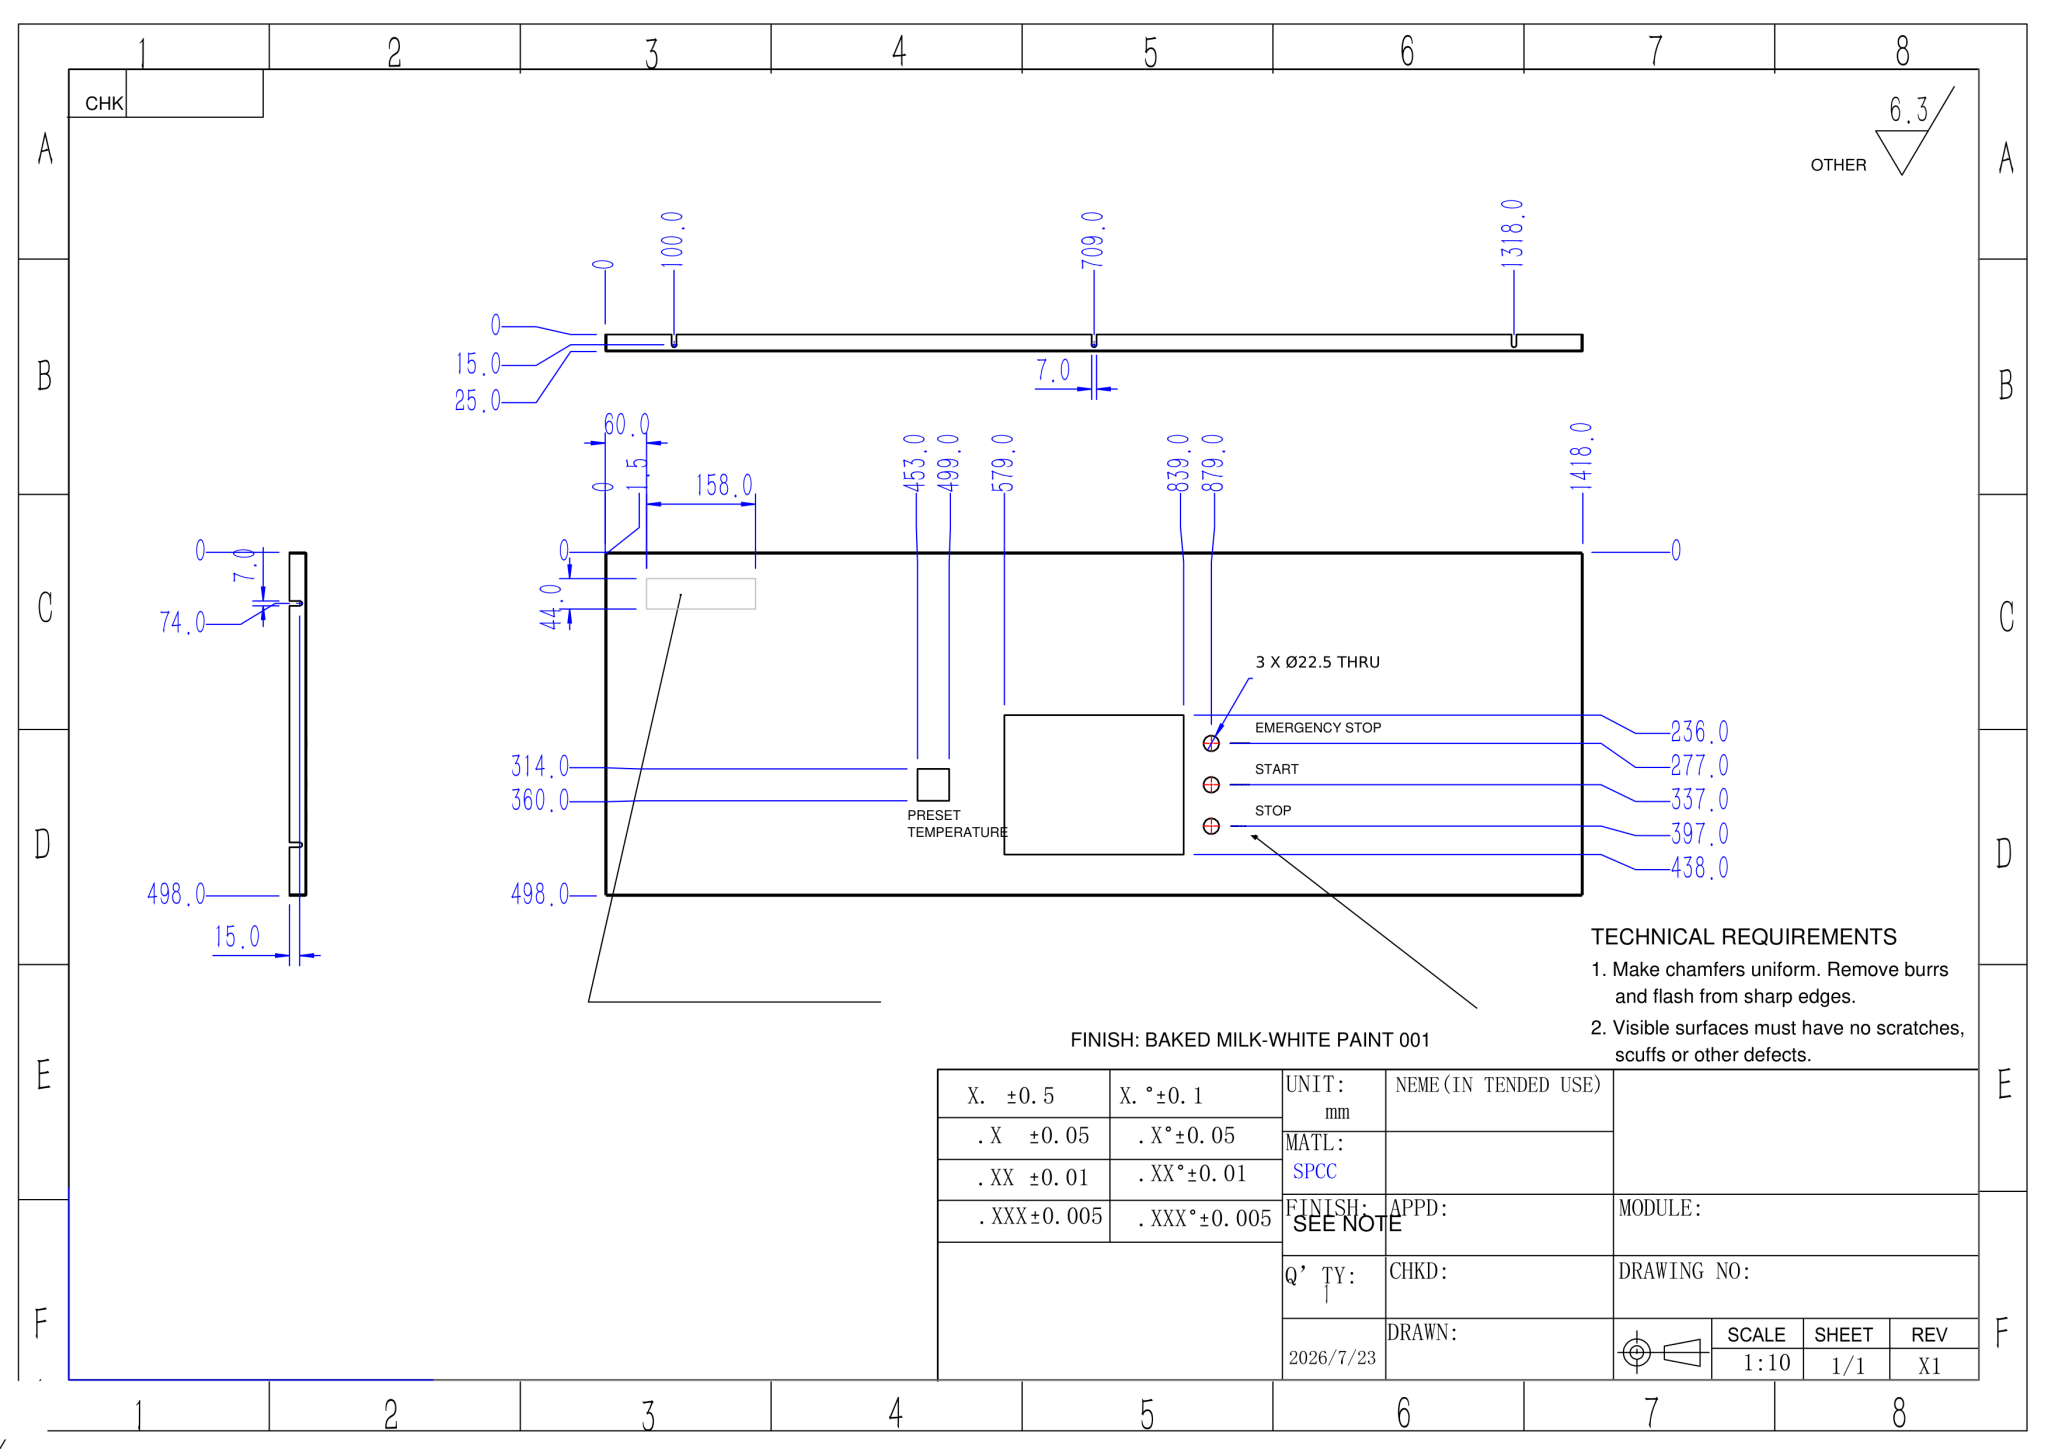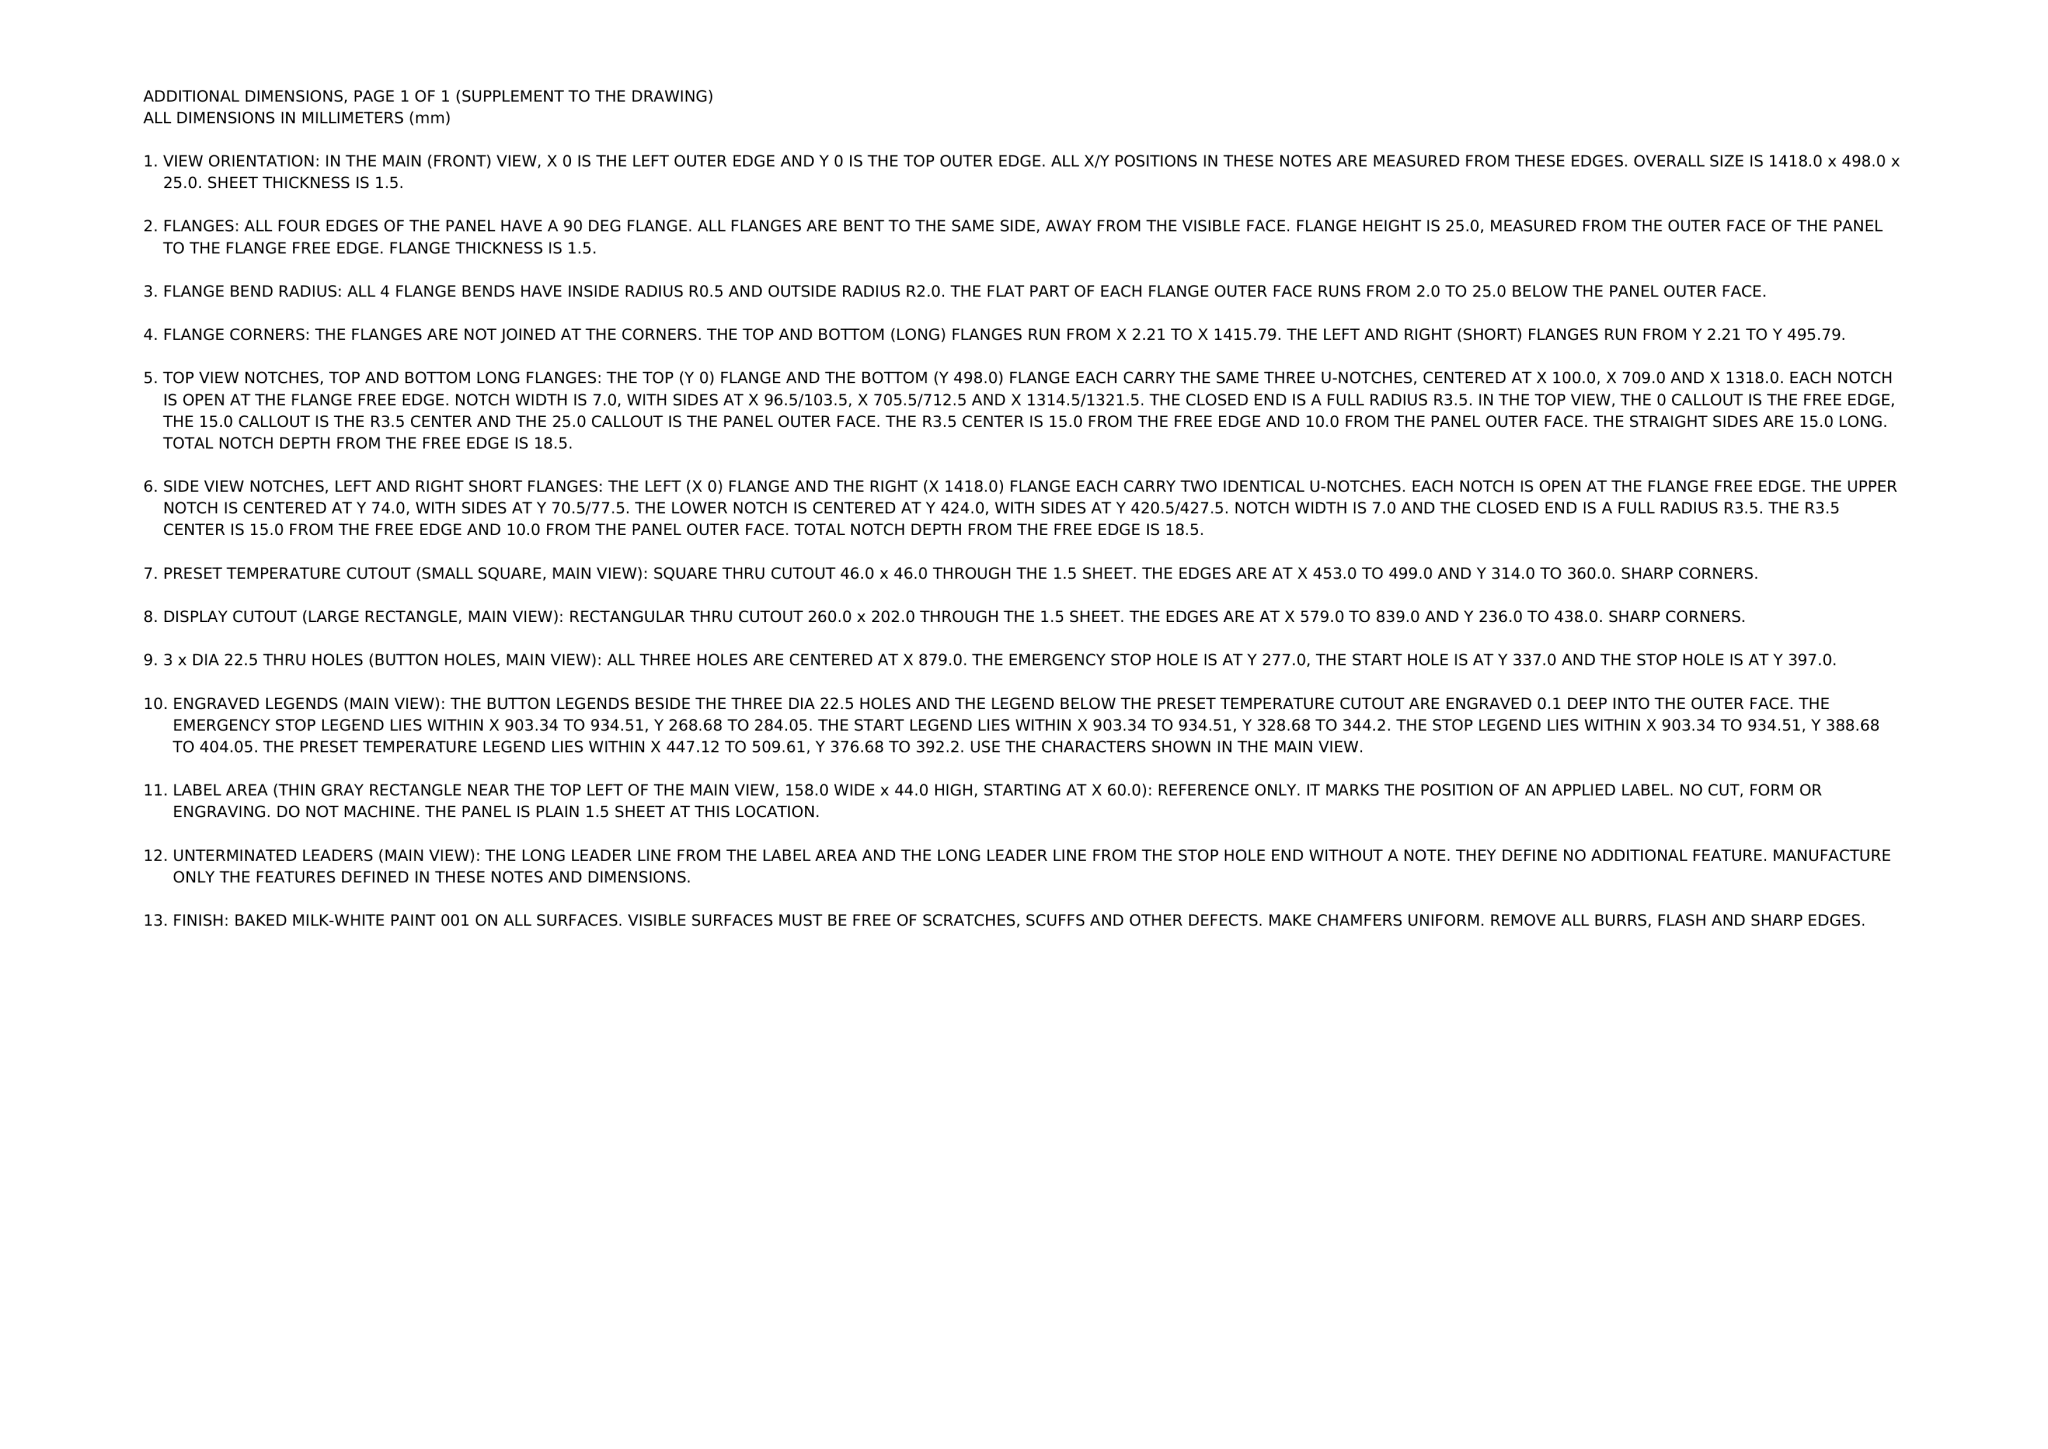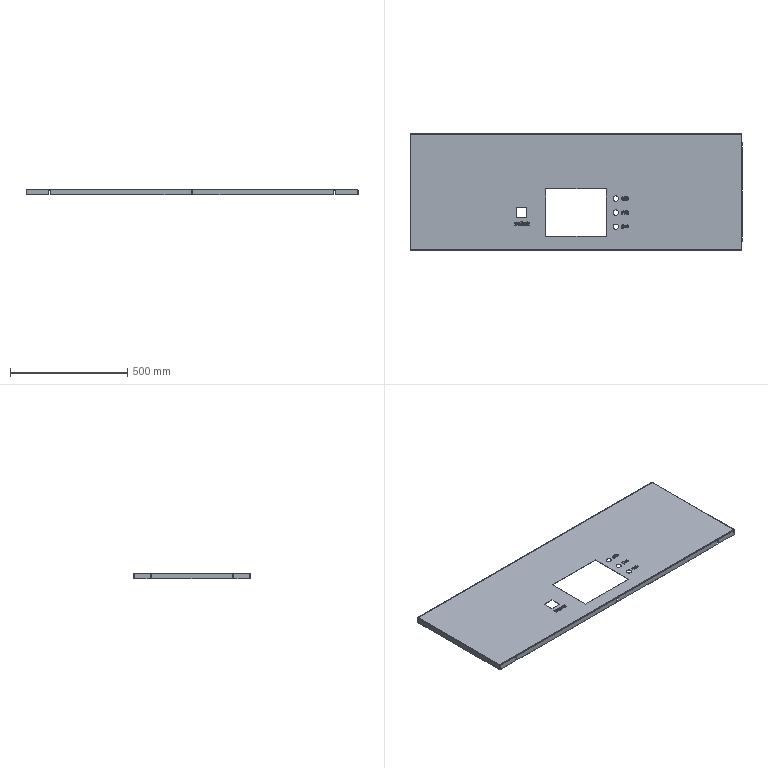Part | NX | mm | 1 solid | 576 faces | box 1418 x 498 x 25 mm | volume 1104917 mm3 | plane 416 | spline 126 | cylinder 34 | commonest cylinder face diameters 7 x20 22.5 x6 4 x4 1 x4